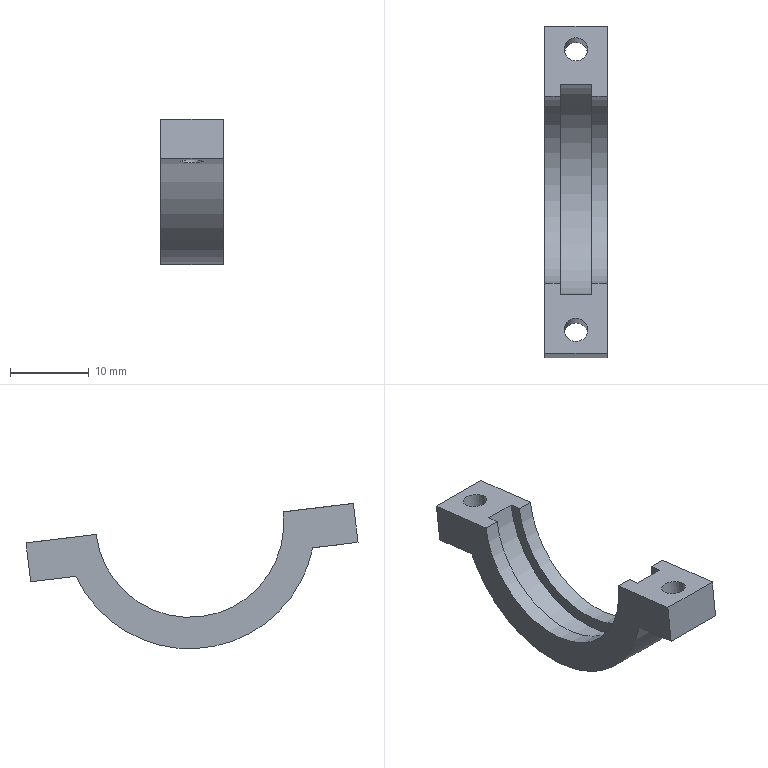Component | NX | 20B__27 | 1 solid | 16 faces | volume 1518 mm3 | plane 10 | cylinder 6 | commonest cylinder face diameters 24 x2 3 x2 32 x1 27 x1